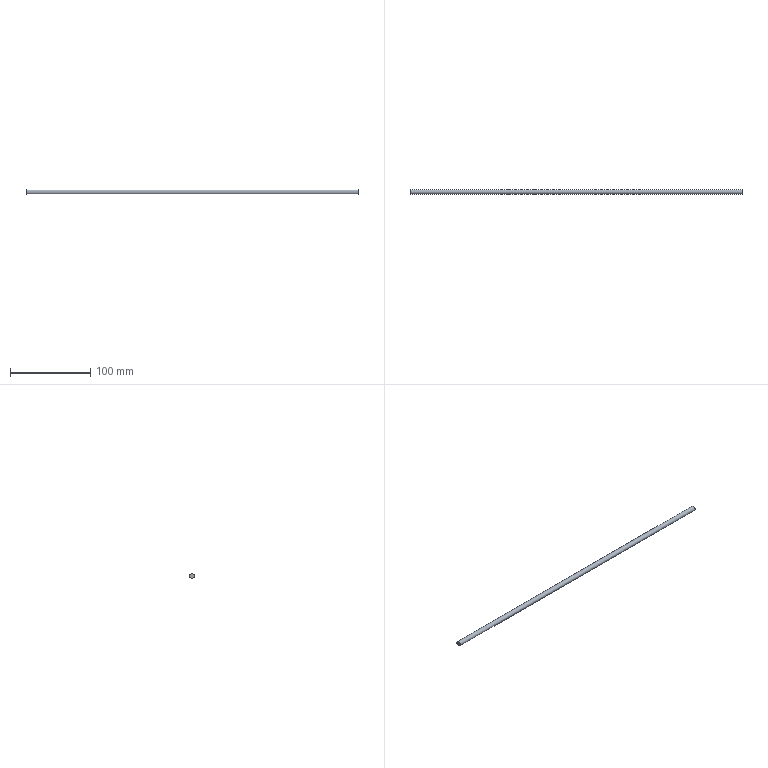Component | NX | LONG_SHAFT | 1 solid | 3 faces | box 414.5 x 6 x 6 mm | volume 11720 mm3 | plane 2 | cylinder 1 | commonest cylinder face diameters 6 x1
STEP:
#1=CARTESIAN_POINT('',(0.,0.,0.));
#2=DIRECTION('',(0.,0.,1.));
#3=DIRECTION('',(1.,0.,0.));
#4=AXIS2_PLACEMENT_3D('',#1,#2,#3);
#5=CARTESIAN_POINT('',(207.25,44.316,20.));
#6=VERTEX_POINT('',#5);
#7=CARTESIAN_POINT('',(207.25,41.316,20.));
#8=DIRECTION('',(1.,0.,-0.));
#9=DIRECTION('',(-0.,1.,0.));
#10=AXIS2_PLACEMENT_3D('',#7,#8,#9);
#11=CIRCLE('',#10,3.);
#12=CARTESIAN_POINT('',(207.25,41.316,20.));
#13=DIRECTION('',(-1.,0.,0.));
#14=DIRECTION('',(0.,0.04536,0.999));
#15=AXIS2_PLACEMENT_3D('',#12,#13,#14);
#16=CYLINDRICAL_SURFACE('',#15,3.);
#17=CARTESIAN_POINT('',(7.809,0.));
#18=DIRECTION('',(-1.,0.));
#19=VECTOR('',#18,1.);
#20=LINE('',#17,#19);
#21=(GEOMETRIC_REPRESENTATION_CONTEXT(2)PARAMETRIC_REPRESENTATION_CONTEXT()REPRESENTATION_CONTEXT('',''));
#22=DEFINITIONAL_REPRESENTATION('',(#20),#21);
#23=PCURVE('',#16,#22);
#24=CARTESIAN_POINT('',(207.25,41.316,20.));
#25=DIRECTION('',(1.,0.,-0.));
#26=DIRECTION('',(-0.,0.999,-0.04536));
#27=AXIS2_PLACEMENT_3D('',#24,#25,#26);
#28=PLANE('',#27);
#29=CARTESIAN_POINT('',(0.,0.));
#30=DIRECTION('',(0.999,0.04536));
#31=AXIS2_PLACEMENT_2D('',#29,#30);
#32=CIRCLE('',#31,3.);
#33=(GEOMETRIC_REPRESENTATION_CONTEXT(2)PARAMETRIC_REPRESENTATION_CONTEXT()REPRESENTATION_CONTEXT('',''));
#34=DEFINITIONAL_REPRESENTATION('',(#32),#33);
#35=PCURVE('',#28,#34);
#36=SURFACE_CURVE('',#11,(#23,#35),.PCURVE_S1.);
#37=EDGE_CURVE('',#6,#6,#36,.T.);
#38=ORIENTED_EDGE('',*,*,#37,.F.);
#39=CARTESIAN_POINT('',(-207.25,44.316,20.));
#40=VERTEX_POINT('',#39);
#41=CARTESIAN_POINT('',(207.25,44.316,20.));
#42=CARTESIAN_POINT('',(-207.25,44.316,20.));
#43=B_SPLINE_CURVE_WITH_KNOTS('',1,(#41,#42),.UNSPECIFIED.,.F.,.F.,(2,2),(0.,414.5),.PIECEWISE_BEZIER_KNOTS.);
#44=CARTESIAN_POINT('',(7.809,0.));
#45=DIRECTION('',(0.,1.));
#46=VECTOR('',#45,1.);
#47=LINE('',#44,#46);
#48=(GEOMETRIC_REPRESENTATION_CONTEXT(2)PARAMETRIC_REPRESENTATION_CONTEXT()REPRESENTATION_CONTEXT('',''));
#49=DEFINITIONAL_REPRESENTATION('',(#47),#48);
#50=PCURVE('',#16,#49);
#51=CARTESIAN_POINT('',(1.525,0.));
#52=DIRECTION('',(0.,1.));
#53=VECTOR('',#52,1.);
#54=LINE('',#51,#53);
#55=(GEOMETRIC_REPRESENTATION_CONTEXT(2)PARAMETRIC_REPRESENTATION_CONTEXT()REPRESENTATION_CONTEXT('',''));
#56=DEFINITIONAL_REPRESENTATION('',(#54),#55);
#57=PCURVE('',#16,#56);
#58=SEAM_CURVE('',#43,(#50,#57),.PCURVE_S1.);
#59=EDGE_CURVE('',#6,#40,#58,.T.);
#60=ORIENTED_EDGE('',*,*,#59,.T.);
#61=CARTESIAN_POINT('',(-207.25,41.316,20.));
#62=DIRECTION('',(1.,0.,-0.));
#63=DIRECTION('',(-0.,1.,0.));
#64=AXIS2_PLACEMENT_3D('',#61,#62,#63);
#65=CIRCLE('',#64,3.);
#66=CARTESIAN_POINT('',(7.809,414.5));
#67=DIRECTION('',(-1.,0.));
#68=VECTOR('',#67,1.);
#69=LINE('',#66,#68);
#70=(GEOMETRIC_REPRESENTATION_CONTEXT(2)PARAMETRIC_REPRESENTATION_CONTEXT()REPRESENTATION_CONTEXT('',''));
#71=DEFINITIONAL_REPRESENTATION('',(#69),#70);
#72=PCURVE('',#16,#71);
#73=CARTESIAN_POINT('',(-207.25,41.316,20.));
#74=DIRECTION('',(1.,0.,-0.));
#75=DIRECTION('',(-0.,0.999,-0.04536));
#76=AXIS2_PLACEMENT_3D('',#73,#74,#75);
#77=PLANE('',#76);
#78=CARTESIAN_POINT('',(0.,0.));
#79=DIRECTION('',(0.999,0.04536));
#80=AXIS2_PLACEMENT_2D('',#78,#79);
#81=CIRCLE('',#80,3.);
#82=(GEOMETRIC_REPRESENTATION_CONTEXT(2)PARAMETRIC_REPRESENTATION_CONTEXT()REPRESENTATION_CONTEXT('',''));
#83=DEFINITIONAL_REPRESENTATION('',(#81),#82);
#84=PCURVE('',#77,#83);
#85=SURFACE_CURVE('',#65,(#72,#84),.PCURVE_S1.);
#86=EDGE_CURVE('',#40,#40,#85,.T.);
#87=ORIENTED_EDGE('',*,*,#86,.T.);
#88=ORIENTED_EDGE('',*,*,#59,.F.);
#89=EDGE_LOOP('',(#38,#60,#87,#88));
#90=FACE_BOUND('',#89,.T.);
#91=ADVANCED_FACE('',(#90),#16,.T.);
#92=ORIENTED_EDGE('',*,*,#37,.T.);
#93=EDGE_LOOP('',(#92));
#94=FACE_BOUND('',#93,.T.);
#95=ADVANCED_FACE('',(#94),#28,.T.);
#96=ORIENTED_EDGE('',*,*,#86,.F.);
#97=EDGE_LOOP('',(#96));
#98=FACE_BOUND('',#97,.T.);
#99=ADVANCED_FACE('',(#98),#77,.F.);
#100=CLOSED_SHELL('',(#91,#95,#99));
#101=MANIFOLD_SOLID_BREP('',#100);
#102=(LENGTH_UNIT()NAMED_UNIT(*)SI_UNIT(.MILLI.,.METRE.));
#103=UNCERTAINTY_MEASURE_WITH_UNIT(LENGTH_MEASURE(0.00001),#102,'','');
#104=(NAMED_UNIT(*)PLANE_ANGLE_UNIT()SI_UNIT($,.RADIAN.));
#105=(NAMED_UNIT(*)SI_UNIT($,.STERADIAN.)SOLID_ANGLE_UNIT());
#106=(GEOMETRIC_REPRESENTATION_CONTEXT(3)GLOBAL_UNCERTAINTY_ASSIGNED_CONTEXT((#103))GLOBAL_UNIT_ASSIGNED_CONTEXT((#102,#104,#105))REPRESENTATION_CONTEXT('',''));
#107=ADVANCED_BREP_SHAPE_REPRESENTATION('',(#4,#101),#106);